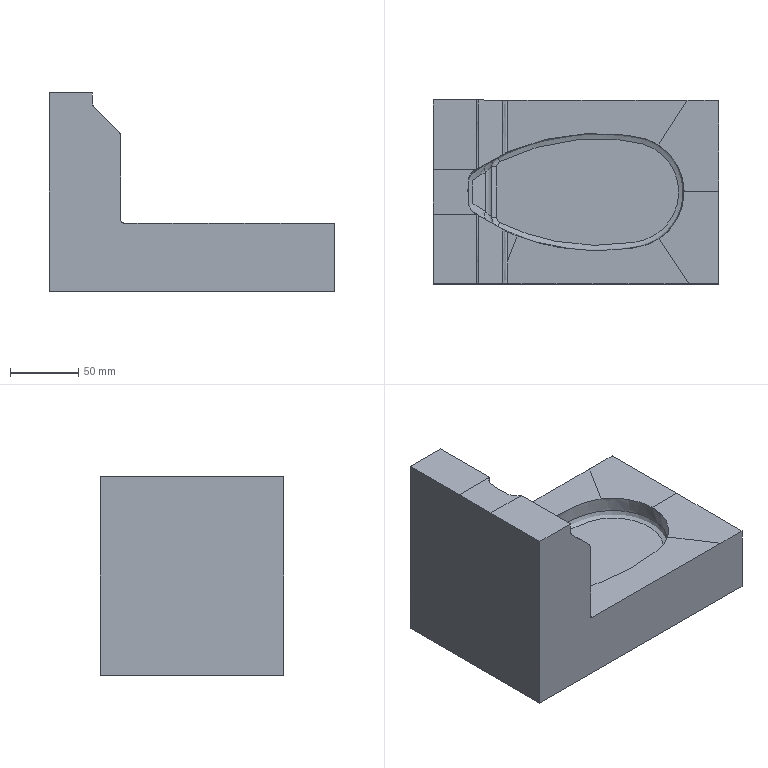CAM job | NX | mm | 3-axis | 1 set-up | 5 operations | part box 210 x 135 x 145.57
set-up 1
1. Cavity Milling | Mill Mill5 D20R4 | CAVITY_MILL | path 1108619.216 mm | 1781.536 min
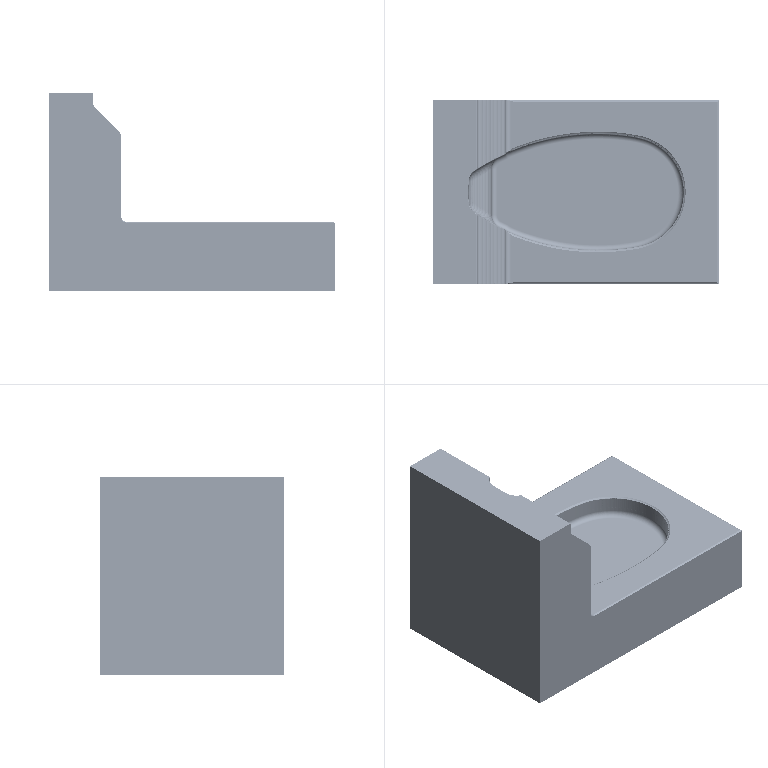2. Volume Based 2.5D Milling | Mill Mill5 D16R1 | FLOOR_WALL | path 2932.084 mm | 10.122 min
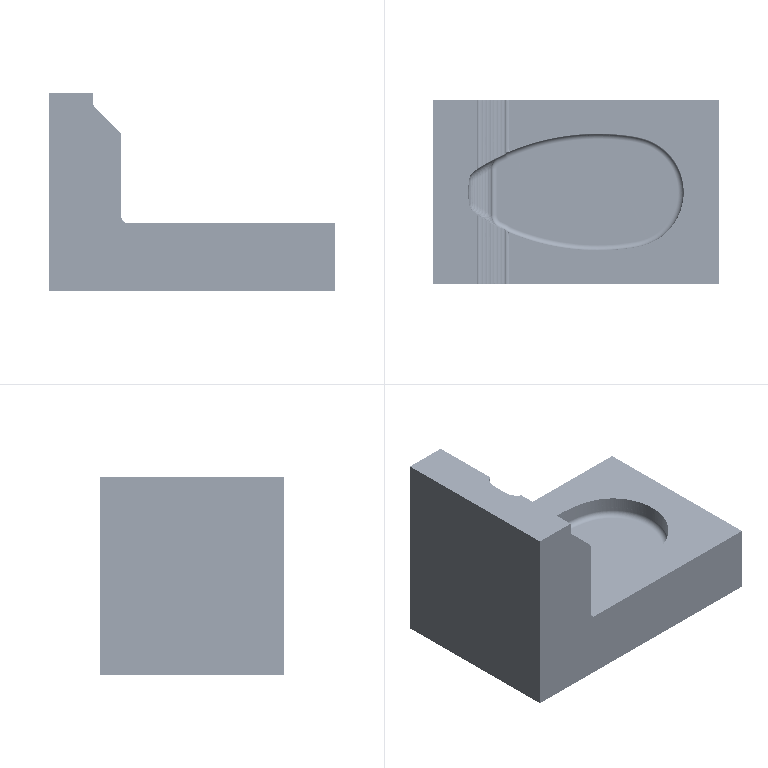3. Volume Based 2.5D Milling | Mill Mill5 D16R1 | FLOOR_WALL_COPY | path 1230.207 mm | 3.937 min
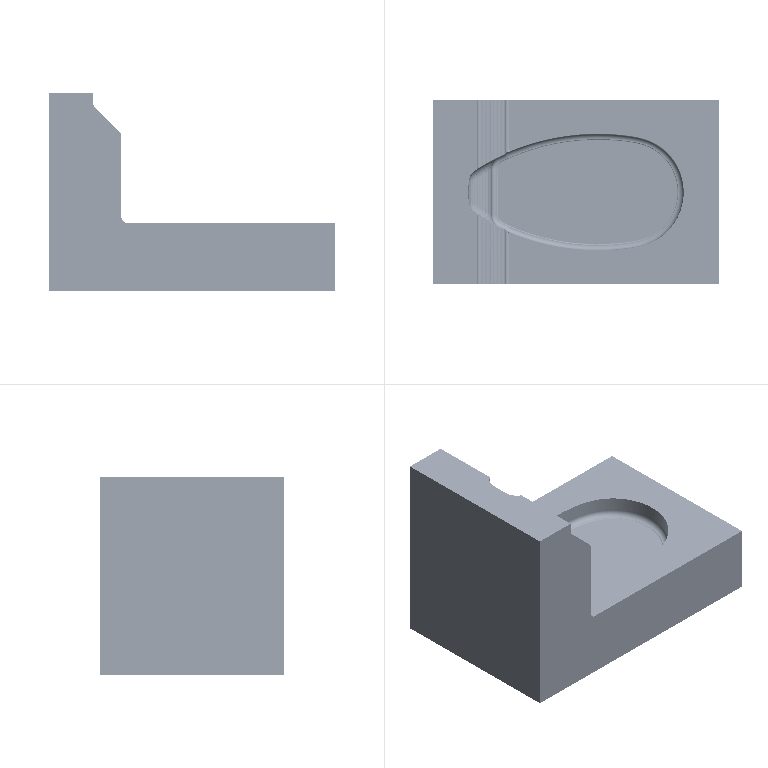4. Z-Level Milling | Mill Mill5 D16R1 | ZLEVEL_PROFILE | path 21343.969 mm | 82.935 min
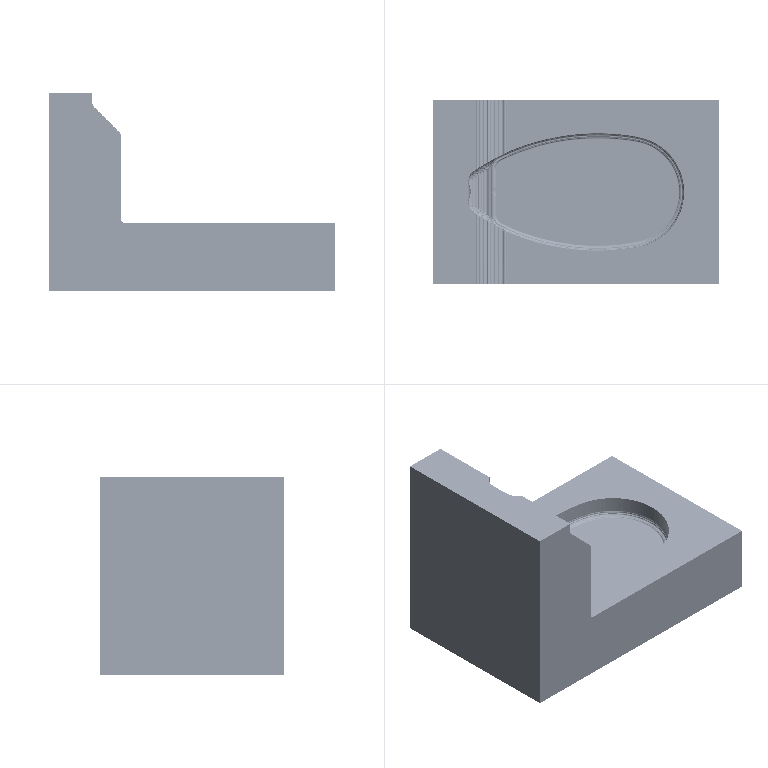5. Fixed-axis Surface Contouring | Mill Mill5 D16R1 | FIXED_CONTOUR | path 5775.213 mm | 22.475 min